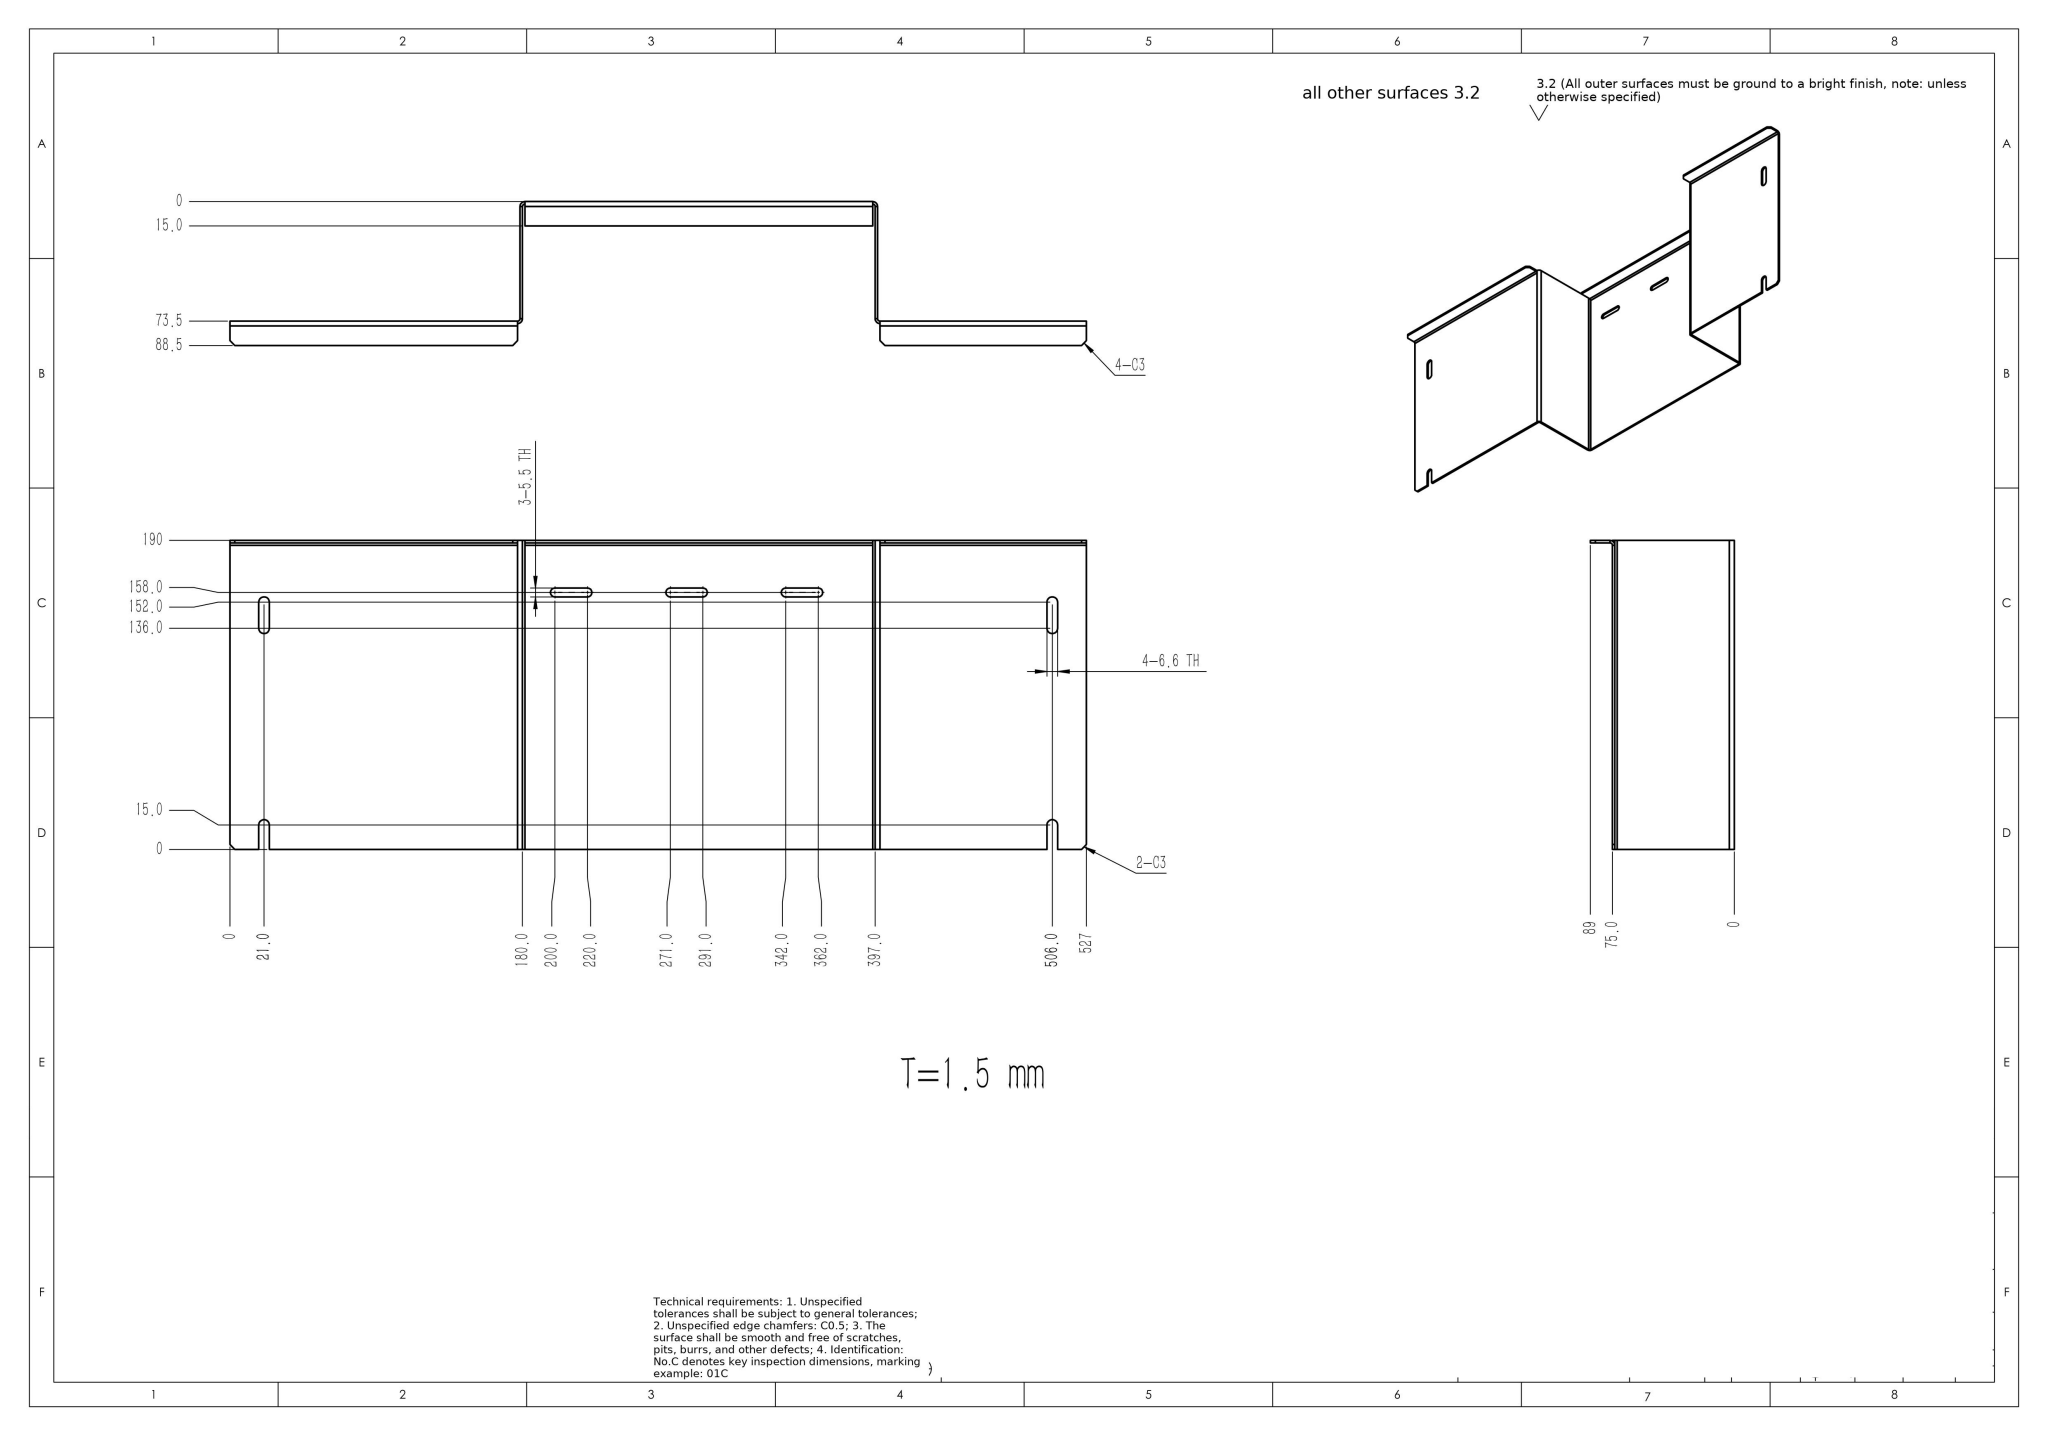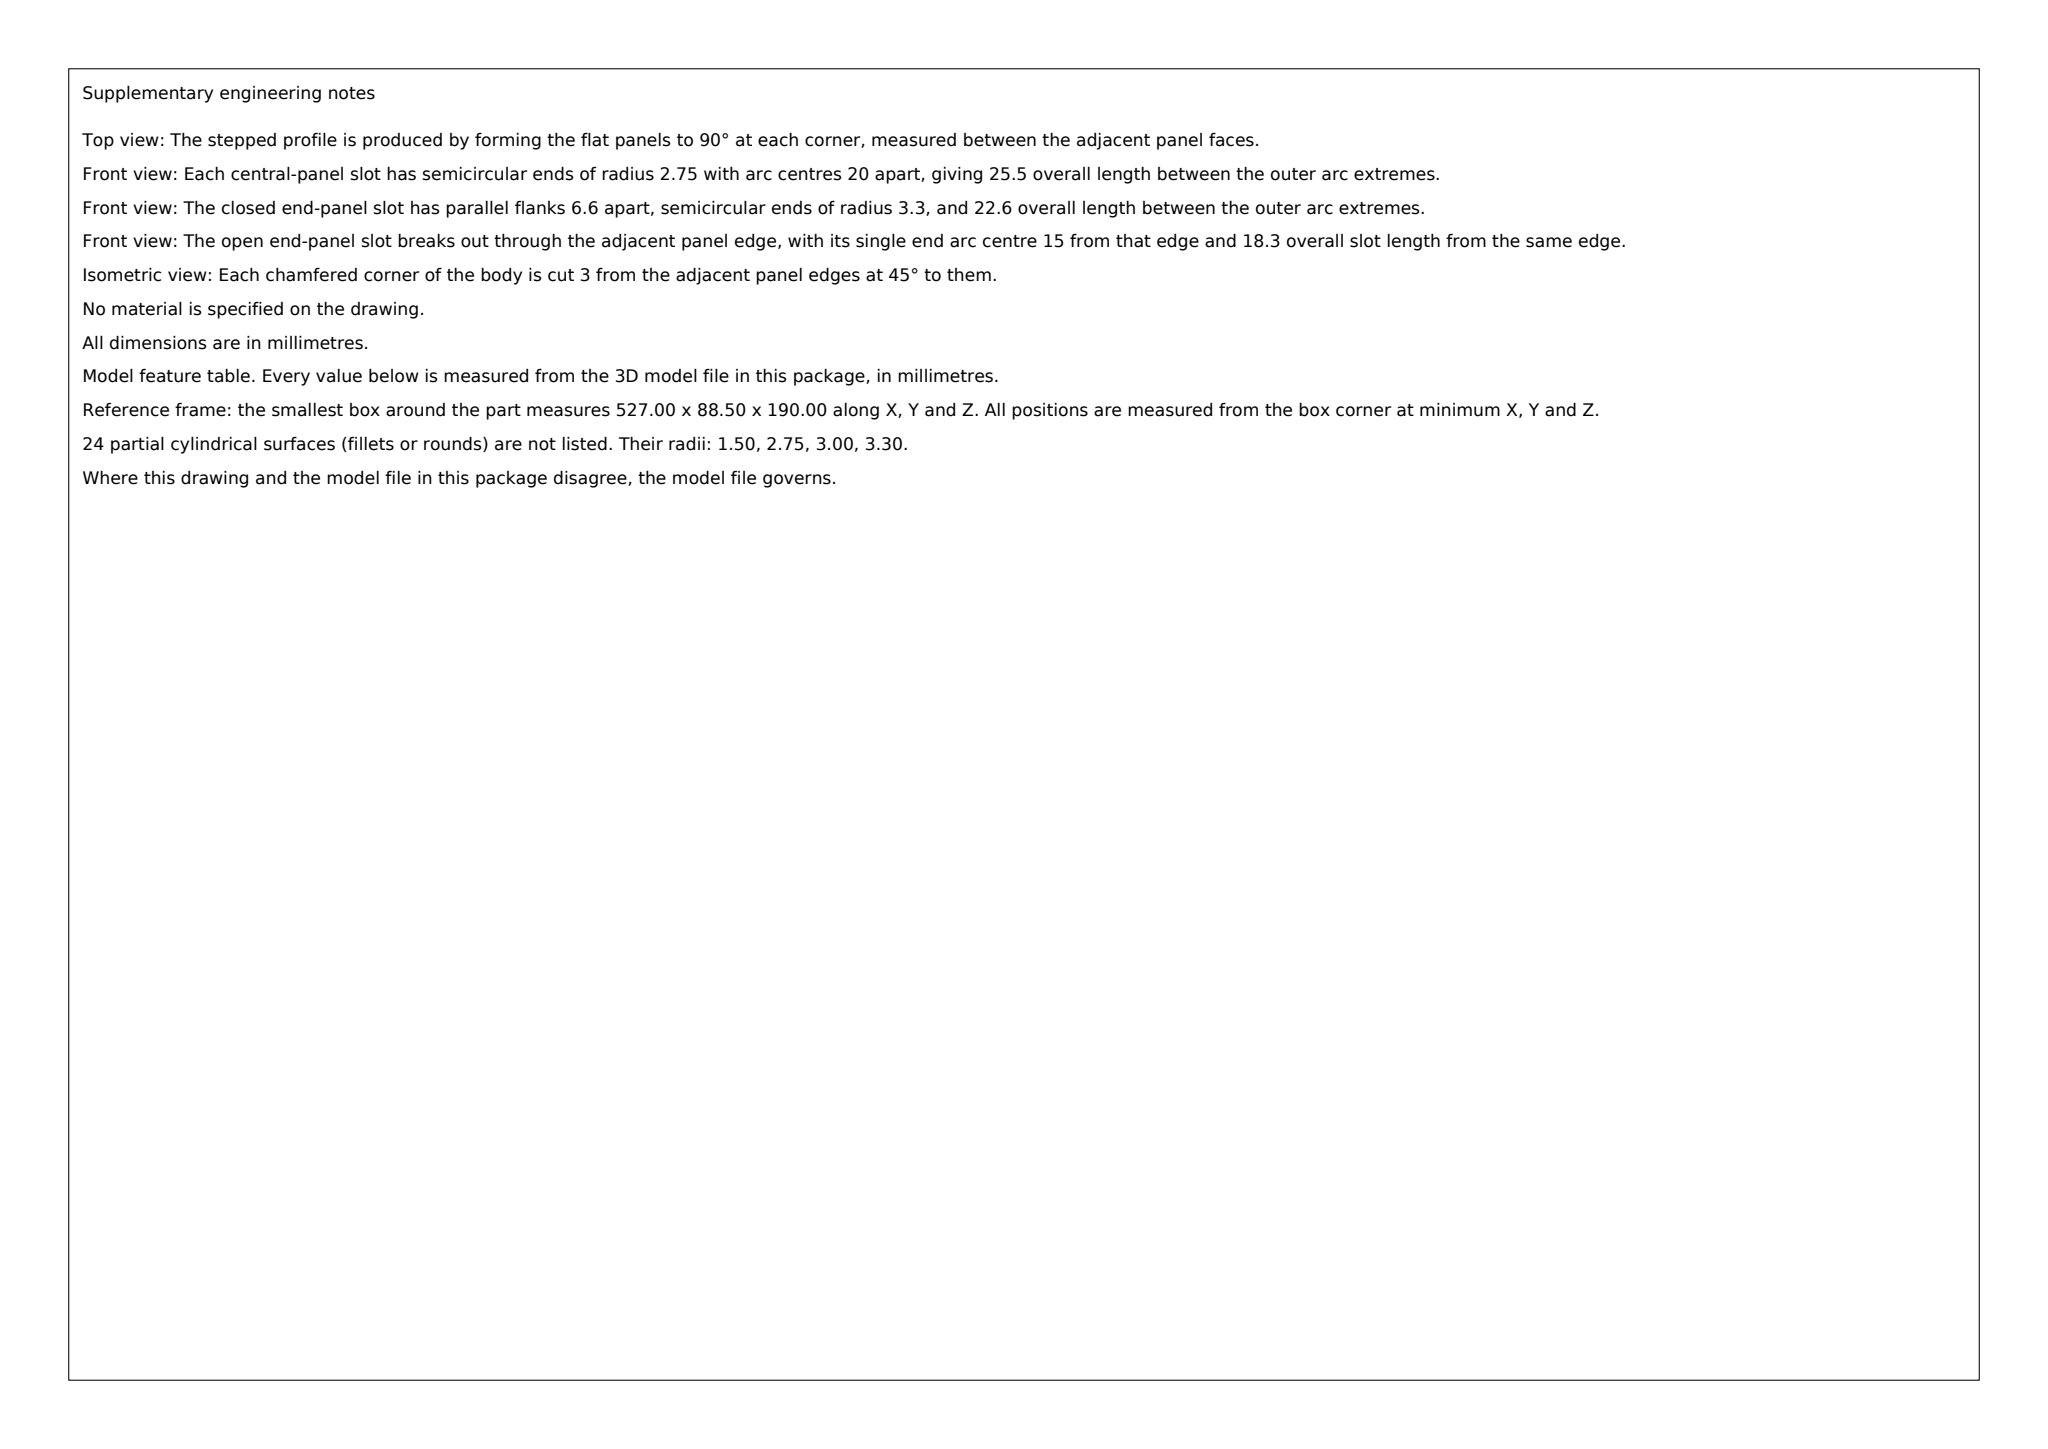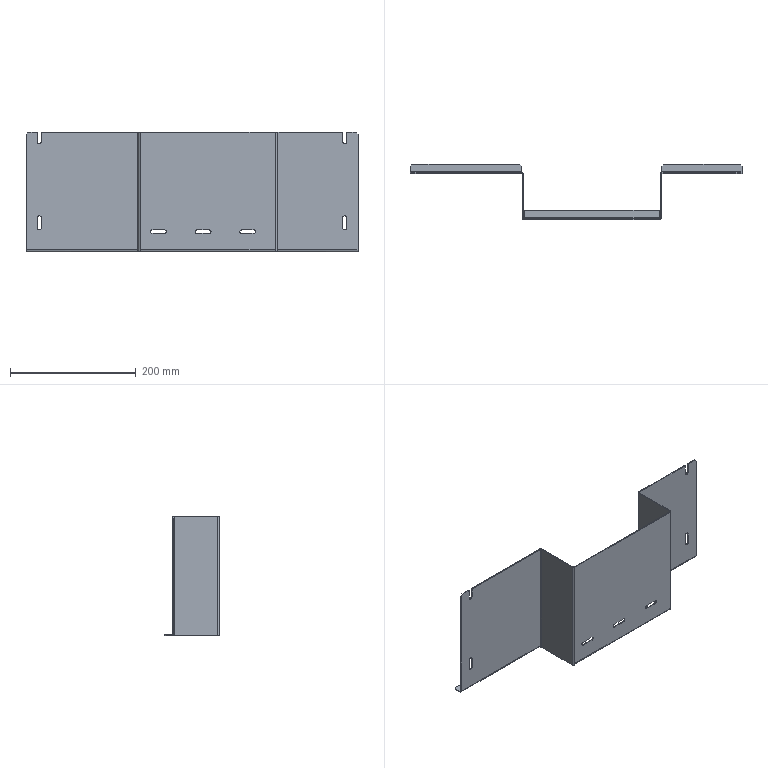Part | SolidWorks | mm | 1 solid | 104 faces | box 527 x 88.5 x 190 mm | volume 199318 mm3 | plane 74 | cylinder 30 | commonest cylinder face diameters 6.6 x10 6 x7 3 x7 5.5 x6
Drawing notes:
3X SLOT 5.5 W x 25.5 LG THRU, CTR DIST 20 (MID FACE) | from the solid: Six 5.5 dia y-axis holes thru 1.5 wall at x=200/220, 271/291, 342/362, z=32 -> 3 slots, 5.5 wide, 20 ctr dist, 25.5 overall
4X SLOT 6.6 W THRU: 2 CLOSED CTRS 16, 2 OPEN TO EDGE | from the solid: 6.6 dia y-axis holes thru 1.5 wall at x=21 & 506, z=38 & 54 (closed slot, 16 ctrs) and z=175 breaking z=190 edge (open slot)
OVERALL DEPTH 88.5 ALL VIEWS (NOT 89); 73.5/75.0 = 1.5 THK FACES | from the solid: bbox_xyz y=88.5; y planes at 0, 1.5, 15.0, 73.5, 75.0, 88.5